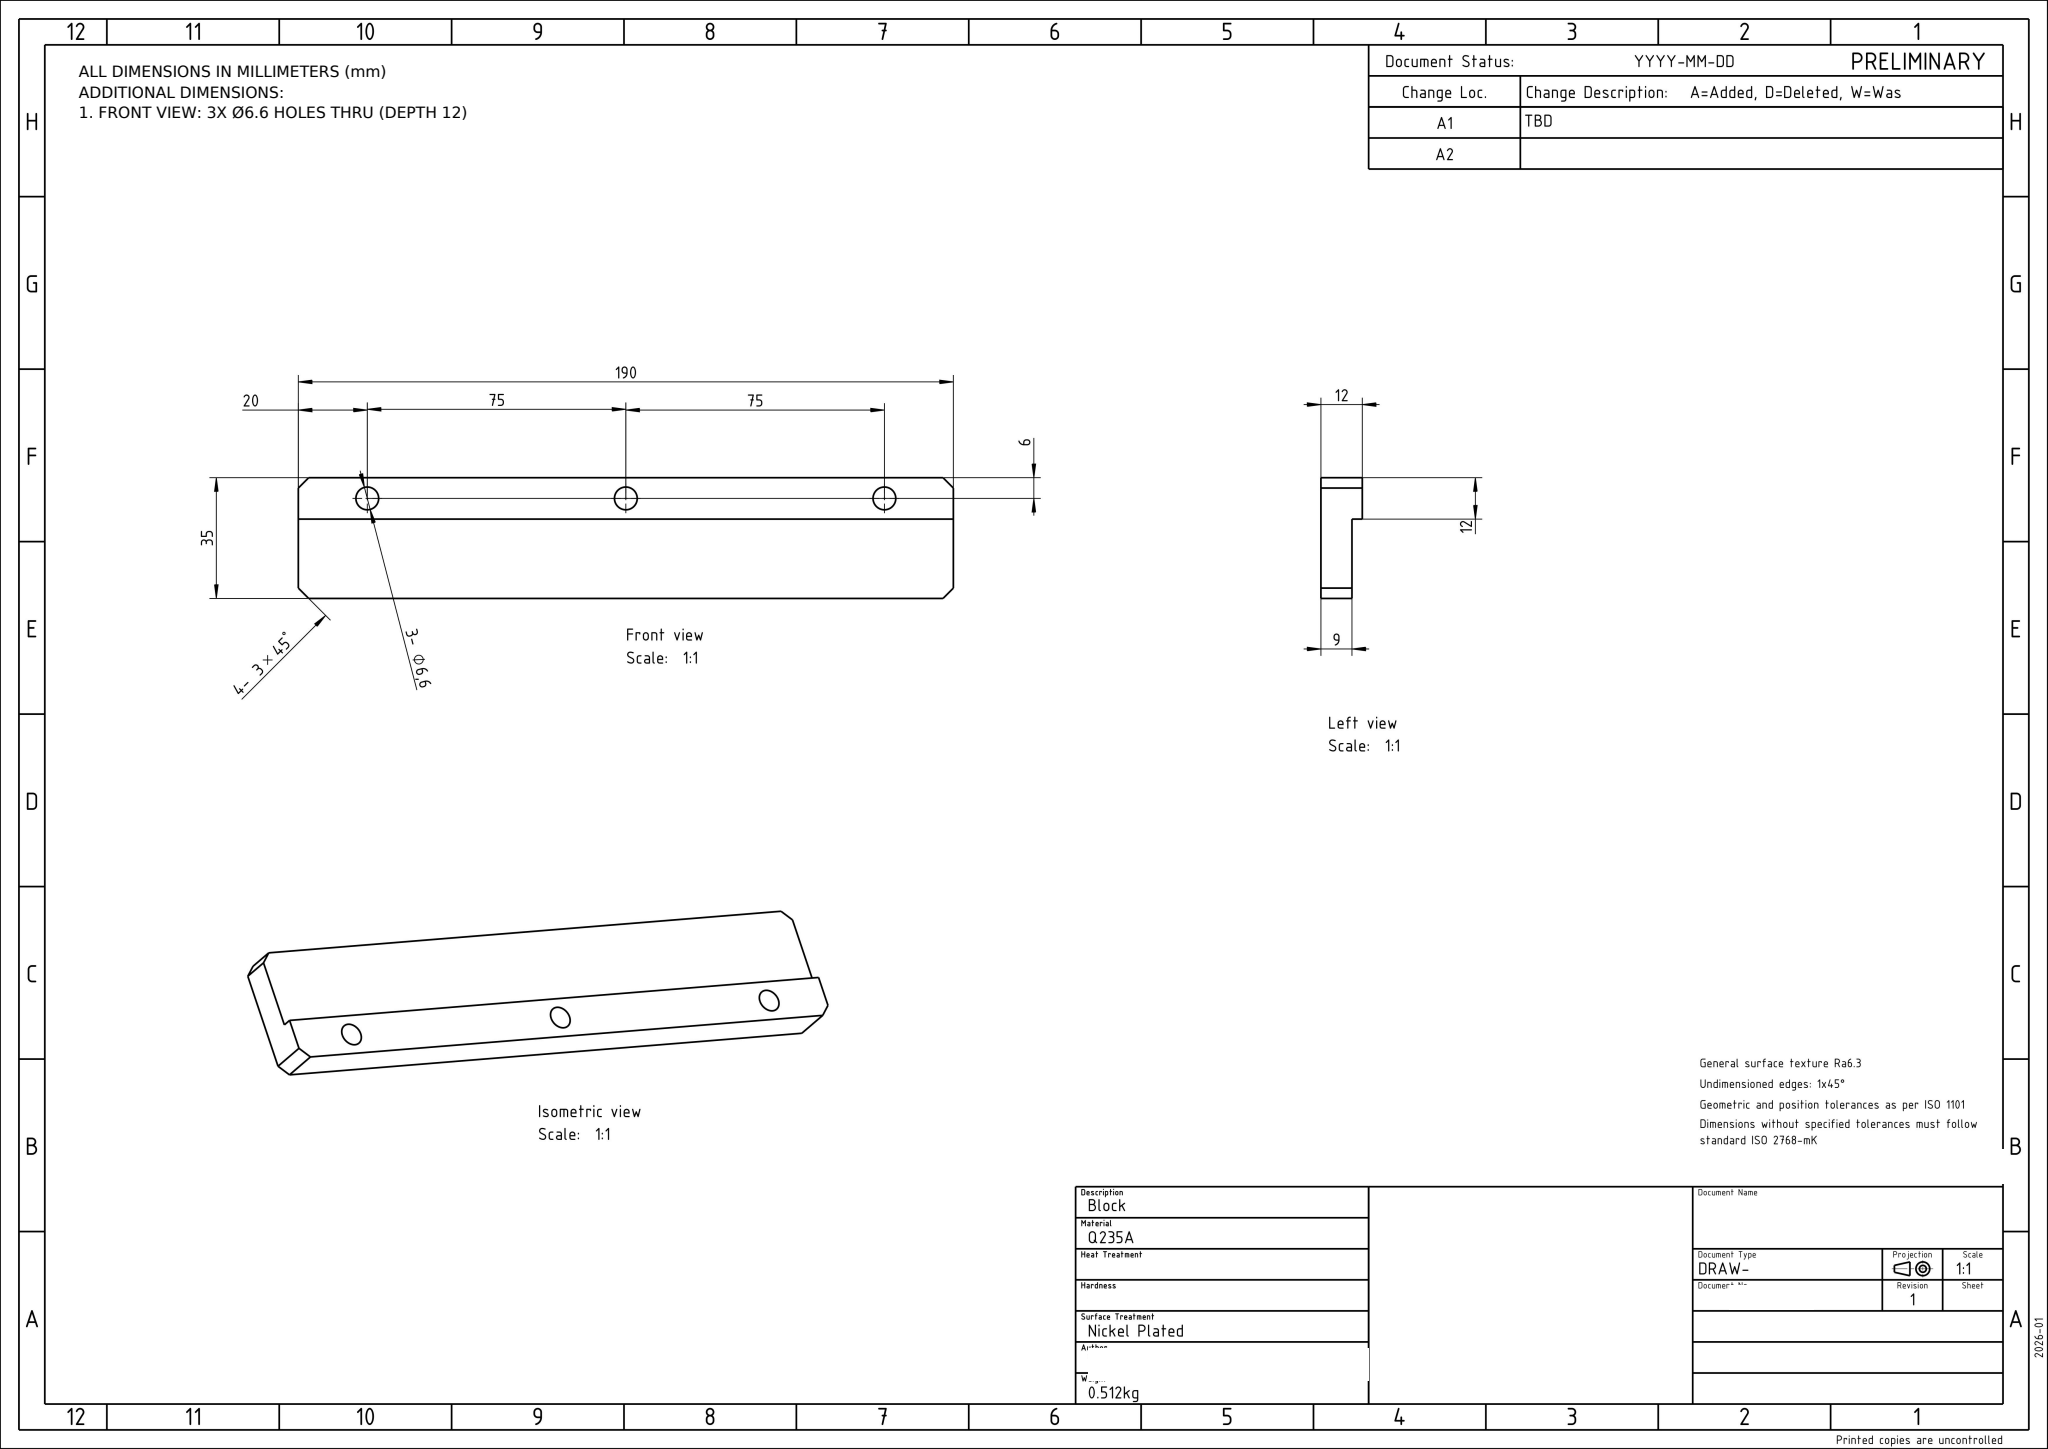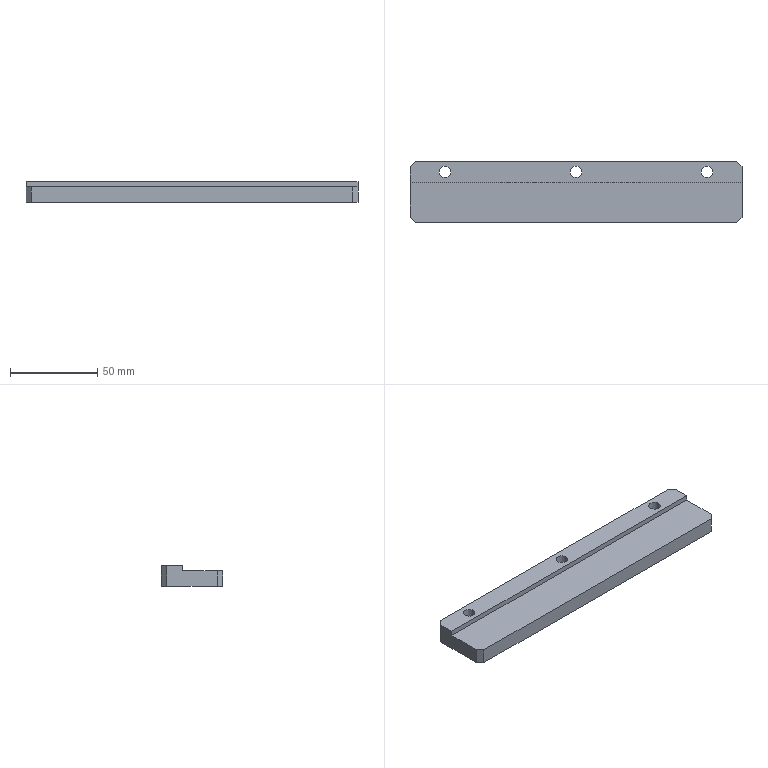Part | NX | mm | 1 solid | 15 faces | box 190 x 35 x 12 mm | volume 65269 mm3 | plane 12 | cylinder 3 | commonest cylinder face diameters 6.6 x3
STEP:
#1=CARTESIAN_POINT('',(0.,0.,0.));
#2=DIRECTION('',(0.,0.,1.));
#3=DIRECTION('',(1.,0.,0.));
#4=AXIS2_PLACEMENT_3D('',#1,#2,#3);
#5=(LENGTH_UNIT()NAMED_UNIT(*)SI_UNIT(.MILLI.,.METRE.));
#6=UNCERTAINTY_MEASURE_WITH_UNIT(LENGTH_MEASURE(0.00002),#5,'','');
#7=(NAMED_UNIT(*)PLANE_ANGLE_UNIT()SI_UNIT($,.RADIAN.));
#8=PLANE_ANGLE_MEASURE_WITH_UNIT(PLANE_ANGLE_MEASURE(0.01745),#7);
#9=DIMENSIONAL_EXPONENTS(0.,0.,0.,0.,0.,0.,0.);
#10=(CONVERSION_BASED_UNIT('',#8)NAMED_UNIT(#9)PLANE_ANGLE_UNIT());
#11=(NAMED_UNIT(*)SI_UNIT($,.STERADIAN.)SOLID_ANGLE_UNIT());
#12=(GEOMETRIC_REPRESENTATION_CONTEXT(3)GLOBAL_UNCERTAINTY_ASSIGNED_CONTEXT((#6))GLOBAL_UNIT_ASSIGNED_CONTEXT((#5,#10,#11))REPRESENTATION_CONTEXT('',''));
#13=SHAPE_REPRESENTATION('',(#4),#12);
#14=CARTESIAN_POINT('',(-95.,14.5,12.));
#15=VERTEX_POINT('',#14);
#16=CARTESIAN_POINT('',(-95.,5.5,12.));
#17=VERTEX_POINT('',#16);
#18=CARTESIAN_POINT('',(-95.,17.5,12.));
#19=DIRECTION('',(0.,-1.,0.));
#20=VECTOR('',#19,1.);
#21=LINE('',#18,#20);
#22=EDGE_CURVE('',#15,#17,#21,.T.);
#23=ORIENTED_EDGE('',*,*,#22,.F.);
#24=CARTESIAN_POINT('',(-95.,14.5,0.));
#25=VERTEX_POINT('',#24);
#26=CARTESIAN_POINT('',(-95.,14.5,9.));
#27=DIRECTION('',(0.,0.,-1.));
#28=VECTOR('',#27,1.);
#29=LINE('',#26,#28);
#30=EDGE_CURVE('',#15,#25,#29,.T.);
#31=ORIENTED_EDGE('',*,*,#30,.T.);
#32=CARTESIAN_POINT('',(-95.,-14.5,0.));
#33=VERTEX_POINT('',#32);
#34=CARTESIAN_POINT('',(-95.,17.5,0.));
#35=DIRECTION('',(0.,-1.,0.));
#36=VECTOR('',#35,1.);
#37=LINE('',#34,#36);
#38=EDGE_CURVE('',#25,#33,#37,.T.);
#39=ORIENTED_EDGE('',*,*,#38,.T.);
#40=CARTESIAN_POINT('',(-95.,-14.5,9.));
#41=VERTEX_POINT('',#40);
#42=CARTESIAN_POINT('',(-95.,-14.5,9.));
#43=DIRECTION('',(0.,0.,1.));
#44=VECTOR('',#43,1.);
#45=LINE('',#42,#44);
#46=EDGE_CURVE('',#33,#41,#45,.T.);
#47=ORIENTED_EDGE('',*,*,#46,.T.);
#48=CARTESIAN_POINT('',(-95.,5.5,9.));
#49=VERTEX_POINT('',#48);
#50=CARTESIAN_POINT('',(-95.,17.5,9.));
#51=DIRECTION('',(0.,-1.,0.));
#52=VECTOR('',#51,1.);
#53=LINE('',#50,#52);
#54=EDGE_CURVE('',#49,#41,#53,.T.);
#55=ORIENTED_EDGE('',*,*,#54,.F.);
#56=CARTESIAN_POINT('',(-95.,5.5,9.));
#57=DIRECTION('',(0.,0.,1.));
#58=VECTOR('',#57,1.);
#59=LINE('',#56,#58);
#60=EDGE_CURVE('',#49,#17,#59,.T.);
#61=ORIENTED_EDGE('',*,*,#60,.T.);
#62=EDGE_LOOP('',(#23,#31,#39,#47,#55,#61));
#63=FACE_OUTER_BOUND('',#62,.T.);
#64=CARTESIAN_POINT('',(-95.,17.5,9.));
#65=DIRECTION('',(1.,0.,0.));
#66=DIRECTION('',(-0.,1.,0.));
#67=AXIS2_PLACEMENT_3D('',#64,#65,#66);
#68=PLANE('',#67);
#69=ADVANCED_FACE('',(#63),#68,.F.);
#70=CARTESIAN_POINT('',(-92.,-17.5,0.));
#71=VERTEX_POINT('',#70);
#72=CARTESIAN_POINT('',(92.,-17.5,0.));
#73=VERTEX_POINT('',#72);
#74=CARTESIAN_POINT('',(-95.,-17.5,0.));
#75=DIRECTION('',(1.,0.,0.));
#76=VECTOR('',#75,1.);
#77=LINE('',#74,#76);
#78=EDGE_CURVE('',#71,#73,#77,.T.);
#79=ORIENTED_EDGE('',*,*,#78,.T.);
#80=CARTESIAN_POINT('',(92.,-17.5,9.));
#81=VERTEX_POINT('',#80);
#82=CARTESIAN_POINT('',(92.,-17.5,9.));
#83=DIRECTION('',(0.,0.,1.));
#84=VECTOR('',#83,1.);
#85=LINE('',#82,#84);
#86=EDGE_CURVE('',#73,#81,#85,.T.);
#87=ORIENTED_EDGE('',*,*,#86,.T.);
#88=CARTESIAN_POINT('',(-92.,-17.5,9.));
#89=VERTEX_POINT('',#88);
#90=CARTESIAN_POINT('',(-95.,-17.5,9.));
#91=DIRECTION('',(1.,0.,0.));
#92=VECTOR('',#91,1.);
#93=LINE('',#90,#92);
#94=EDGE_CURVE('',#89,#81,#93,.T.);
#95=ORIENTED_EDGE('',*,*,#94,.F.);
#96=CARTESIAN_POINT('',(-92.,-17.5,9.));
#97=DIRECTION('',(0.,0.,-1.));
#98=VECTOR('',#97,1.);
#99=LINE('',#96,#98);
#100=EDGE_CURVE('',#89,#71,#99,.T.);
#101=ORIENTED_EDGE('',*,*,#100,.T.);
#102=EDGE_LOOP('',(#79,#87,#95,#101));
#103=FACE_OUTER_BOUND('',#102,.T.);
#104=CARTESIAN_POINT('',(-95.,-17.5,9.));
#105=DIRECTION('',(0.,1.,0.));
#106=DIRECTION('',(0.,0.,1.));
#107=AXIS2_PLACEMENT_3D('',#104,#105,#106);
#108=PLANE('',#107);
#109=ADVANCED_FACE('',(#103),#108,.F.);
#110=CARTESIAN_POINT('',(95.,-14.5,0.));
#111=VERTEX_POINT('',#110);
#112=CARTESIAN_POINT('',(95.,14.5,0.));
#113=VERTEX_POINT('',#112);
#114=CARTESIAN_POINT('',(95.,-17.5,0.));
#115=DIRECTION('',(-0.,1.,0.));
#116=VECTOR('',#115,1.);
#117=LINE('',#114,#116);
#118=EDGE_CURVE('',#111,#113,#117,.T.);
#119=ORIENTED_EDGE('',*,*,#118,.T.);
#120=CARTESIAN_POINT('',(95.,14.5,12.));
#121=VERTEX_POINT('',#120);
#122=CARTESIAN_POINT('',(95.,14.5,9.));
#123=DIRECTION('',(0.,0.,1.));
#124=VECTOR('',#123,1.);
#125=LINE('',#122,#124);
#126=EDGE_CURVE('',#113,#121,#125,.T.);
#127=ORIENTED_EDGE('',*,*,#126,.T.);
#128=CARTESIAN_POINT('',(95.,5.5,12.));
#129=VERTEX_POINT('',#128);
#130=CARTESIAN_POINT('',(95.,17.5,12.));
#131=DIRECTION('',(0.,-1.,0.));
#132=VECTOR('',#131,1.);
#133=LINE('',#130,#132);
#134=EDGE_CURVE('',#121,#129,#133,.T.);
#135=ORIENTED_EDGE('',*,*,#134,.T.);
#136=CARTESIAN_POINT('',(95.,5.5,9.));
#137=VERTEX_POINT('',#136);
#138=CARTESIAN_POINT('',(95.,5.5,9.));
#139=DIRECTION('',(0.,0.,1.));
#140=VECTOR('',#139,1.);
#141=LINE('',#138,#140);
#142=EDGE_CURVE('',#137,#129,#141,.T.);
#143=ORIENTED_EDGE('',*,*,#142,.F.);
#144=CARTESIAN_POINT('',(95.,-14.5,9.));
#145=VERTEX_POINT('',#144);
#146=CARTESIAN_POINT('',(95.,-17.5,9.));
#147=DIRECTION('',(-0.,1.,0.));
#148=VECTOR('',#147,1.);
#149=LINE('',#146,#148);
#150=EDGE_CURVE('',#145,#137,#149,.T.);
#151=ORIENTED_EDGE('',*,*,#150,.F.);
#152=CARTESIAN_POINT('',(95.,-14.5,9.));
#153=DIRECTION('',(0.,0.,-1.));
#154=VECTOR('',#153,1.);
#155=LINE('',#152,#154);
#156=EDGE_CURVE('',#145,#111,#155,.T.);
#157=ORIENTED_EDGE('',*,*,#156,.T.);
#158=EDGE_LOOP('',(#119,#127,#135,#143,#151,#157));
#159=FACE_OUTER_BOUND('',#158,.T.);
#160=CARTESIAN_POINT('',(95.,-17.5,9.));
#161=DIRECTION('',(-1.,-0.,0.));
#162=DIRECTION('',(0.,-1.,0.));
#163=AXIS2_PLACEMENT_3D('',#160,#161,#162);
#164=PLANE('',#163);
#165=ADVANCED_FACE('',(#159),#164,.F.);
#166=CARTESIAN_POINT('',(92.,17.5,0.));
#167=VERTEX_POINT('',#166);
#168=CARTESIAN_POINT('',(-92.,17.5,0.));
#169=VERTEX_POINT('',#168);
#170=CARTESIAN_POINT('',(95.,17.5,0.));
#171=DIRECTION('',(-1.,0.,0.));
#172=VECTOR('',#171,1.);
#173=LINE('',#170,#172);
#174=EDGE_CURVE('',#167,#169,#173,.T.);
#175=ORIENTED_EDGE('',*,*,#174,.T.);
#176=CARTESIAN_POINT('',(-92.,17.5,12.));
#177=VERTEX_POINT('',#176);
#178=CARTESIAN_POINT('',(-92.,17.5,9.));
#179=DIRECTION('',(0.,0.,1.));
#180=VECTOR('',#179,1.);
#181=LINE('',#178,#180);
#182=EDGE_CURVE('',#169,#177,#181,.T.);
#183=ORIENTED_EDGE('',*,*,#182,.T.);
#184=CARTESIAN_POINT('',(92.,17.5,12.));
#185=VERTEX_POINT('',#184);
#186=CARTESIAN_POINT('',(-95.,17.5,12.));
#187=DIRECTION('',(1.,0.,0.));
#188=VECTOR('',#187,1.);
#189=LINE('',#186,#188);
#190=EDGE_CURVE('',#177,#185,#189,.T.);
#191=ORIENTED_EDGE('',*,*,#190,.T.);
#192=CARTESIAN_POINT('',(92.,17.5,9.));
#193=DIRECTION('',(0.,0.,-1.));
#194=VECTOR('',#193,1.);
#195=LINE('',#192,#194);
#196=EDGE_CURVE('',#185,#167,#195,.T.);
#197=ORIENTED_EDGE('',*,*,#196,.T.);
#198=EDGE_LOOP('',(#175,#183,#191,#197));
#199=FACE_OUTER_BOUND('',#198,.T.);
#200=CARTESIAN_POINT('',(95.,17.5,9.));
#201=DIRECTION('',(0.,-1.,0.));
#202=DIRECTION('',(0.,0.,-1.));
#203=AXIS2_PLACEMENT_3D('',#200,#201,#202);
#204=PLANE('',#203);
#205=ADVANCED_FACE('',(#199),#204,.F.);
#206=ORIENTED_EDGE('',*,*,#94,.T.);
#207=CARTESIAN_POINT('',(54.75,-54.75,9.));
#208=DIRECTION('',(0.7071,0.7071,0.));
#209=VECTOR('',#208,1.);
#210=LINE('',#207,#209);
#211=EDGE_CURVE('',#81,#145,#210,.T.);
#212=ORIENTED_EDGE('',*,*,#211,.T.);
#213=ORIENTED_EDGE('',*,*,#150,.T.);
#214=CARTESIAN_POINT('',(-95.,5.5,9.));
#215=DIRECTION('',(1.,0.,0.));
#216=VECTOR('',#215,1.);
#217=LINE('',#214,#216);
#218=EDGE_CURVE('',#49,#137,#217,.T.);
#219=ORIENTED_EDGE('',*,*,#218,.F.);
#220=ORIENTED_EDGE('',*,*,#54,.T.);
#221=CARTESIAN_POINT('',(-54.75,-54.75,9.));
#222=DIRECTION('',(0.7071,-0.7071,0.));
#223=VECTOR('',#222,1.);
#224=LINE('',#221,#223);
#225=EDGE_CURVE('',#41,#89,#224,.T.);
#226=ORIENTED_EDGE('',*,*,#225,.T.);
#227=EDGE_LOOP('',(#206,#212,#213,#219,#220,#226));
#228=FACE_OUTER_BOUND('',#227,.T.);
#229=CARTESIAN_POINT('',(0.,0.,9.));
#230=DIRECTION('',(0.,0.,1.));
#231=DIRECTION('',(1.,0.,0.));
#232=AXIS2_PLACEMENT_3D('',#229,#230,#231);
#233=PLANE('',#232);
#234=ADVANCED_FACE('',(#228),#233,.T.);
#235=CARTESIAN_POINT('',(78.3,11.5,0.));
#236=VERTEX_POINT('',#235);
#237=CARTESIAN_POINT('',(75.,11.5,0.));
#238=DIRECTION('',(0.,0.,1.));
#239=DIRECTION('',(1.,0.,0.));
#240=AXIS2_PLACEMENT_3D('',#237,#238,#239);
#241=CIRCLE('',#240,3.3);
#242=EDGE_CURVE('',#236,#236,#241,.T.);
#243=ORIENTED_EDGE('',*,*,#242,.T.);
#244=EDGE_LOOP('',(#243));
#245=FACE_BOUND('',#244,.T.);
#246=CARTESIAN_POINT('',(3.3,11.5,0.));
#247=VERTEX_POINT('',#246);
#248=CARTESIAN_POINT('',(0.,11.5,0.));
#249=DIRECTION('',(0.,0.,1.));
#250=DIRECTION('',(1.,0.,0.));
#251=AXIS2_PLACEMENT_3D('',#248,#249,#250);
#252=CIRCLE('',#251,3.3);
#253=EDGE_CURVE('',#247,#247,#252,.T.);
#254=ORIENTED_EDGE('',*,*,#253,.T.);
#255=EDGE_LOOP('',(#254));
#256=FACE_BOUND('',#255,.T.);
#257=CARTESIAN_POINT('',(-71.7,11.5,0.));
#258=VERTEX_POINT('',#257);
#259=CARTESIAN_POINT('',(-75.,11.5,0.));
#260=DIRECTION('',(0.,0.,1.));
#261=DIRECTION('',(1.,0.,0.));
#262=AXIS2_PLACEMENT_3D('',#259,#260,#261);
#263=CIRCLE('',#262,3.3);
#264=EDGE_CURVE('',#258,#258,#263,.T.);
#265=ORIENTED_EDGE('',*,*,#264,.T.);
#266=EDGE_LOOP('',(#265));
#267=FACE_BOUND('',#266,.T.);
#268=ORIENTED_EDGE('',*,*,#38,.F.);
#269=CARTESIAN_POINT('',(-95.,14.5,0.));
#270=DIRECTION('',(0.7071,0.7071,0.));
#271=VECTOR('',#270,1.);
#272=LINE('',#269,#271);
#273=EDGE_CURVE('',#25,#169,#272,.T.);
#274=ORIENTED_EDGE('',*,*,#273,.T.);
#275=ORIENTED_EDGE('',*,*,#174,.F.);
#276=CARTESIAN_POINT('',(92.,17.5,0.));
#277=DIRECTION('',(0.7071,-0.7071,0.));
#278=VECTOR('',#277,1.);
#279=LINE('',#276,#278);
#280=EDGE_CURVE('',#167,#113,#279,.T.);
#281=ORIENTED_EDGE('',*,*,#280,.T.);
#282=ORIENTED_EDGE('',*,*,#118,.F.);
#283=CARTESIAN_POINT('',(95.,-14.5,0.));
#284=DIRECTION('',(-0.7071,-0.7071,0.));
#285=VECTOR('',#284,1.);
#286=LINE('',#283,#285);
#287=EDGE_CURVE('',#111,#73,#286,.T.);
#288=ORIENTED_EDGE('',*,*,#287,.T.);
#289=ORIENTED_EDGE('',*,*,#78,.F.);
#290=CARTESIAN_POINT('',(-92.,-17.5,0.));
#291=DIRECTION('',(-0.7071,0.7071,0.));
#292=VECTOR('',#291,1.);
#293=LINE('',#290,#292);
#294=EDGE_CURVE('',#71,#33,#293,.T.);
#295=ORIENTED_EDGE('',*,*,#294,.T.);
#296=EDGE_LOOP('',(#268,#274,#275,#281,#282,#288,#289,#295));
#297=FACE_BOUND('',#296,.T.);
#298=CARTESIAN_POINT('',(0.,0.,0.));
#299=DIRECTION('',(0.,0.,1.));
#300=DIRECTION('',(1.,0.,0.));
#301=AXIS2_PLACEMENT_3D('',#298,#299,#300);
#302=PLANE('',#301);
#303=ADVANCED_FACE('',(#245,#256,#267,#297),#302,.F.);
#304=CARTESIAN_POINT('',(71.7,11.5,12.));
#305=VERTEX_POINT('',#304);
#306=CARTESIAN_POINT('',(75.,11.5,12.));
#307=DIRECTION('',(0.,0.,-1.));
#308=DIRECTION('',(-1.,0.,0.));
#309=AXIS2_PLACEMENT_3D('',#306,#307,#308);
#310=CIRCLE('',#309,3.3);
#311=EDGE_CURVE('',#305,#305,#310,.T.);
#312=ORIENTED_EDGE('',*,*,#311,.T.);
#313=EDGE_LOOP('',(#312));
#314=FACE_BOUND('',#313,.T.);
#315=CARTESIAN_POINT('',(-3.3,11.5,12.));
#316=VERTEX_POINT('',#315);
#317=CARTESIAN_POINT('',(0.,11.5,12.));
#318=DIRECTION('',(0.,0.,-1.));
#319=DIRECTION('',(-1.,0.,0.));
#320=AXIS2_PLACEMENT_3D('',#317,#318,#319);
#321=CIRCLE('',#320,3.3);
#322=EDGE_CURVE('',#316,#316,#321,.T.);
#323=ORIENTED_EDGE('',*,*,#322,.T.);
#324=EDGE_LOOP('',(#323));
#325=FACE_BOUND('',#324,.T.);
#326=CARTESIAN_POINT('',(-78.3,11.5,12.));
#327=VERTEX_POINT('',#326);
#328=CARTESIAN_POINT('',(-75.,11.5,12.));
#329=DIRECTION('',(0.,0.,-1.));
#330=DIRECTION('',(-1.,0.,0.));
#331=AXIS2_PLACEMENT_3D('',#328,#329,#330);
#332=CIRCLE('',#331,3.3);
#333=EDGE_CURVE('',#327,#327,#332,.T.);
#334=ORIENTED_EDGE('',*,*,#333,.T.);
#335=EDGE_LOOP('',(#334));
#336=FACE_BOUND('',#335,.T.);
#337=ORIENTED_EDGE('',*,*,#190,.F.);
#338=CARTESIAN_POINT('',(-93.5,16.,12.));
#339=DIRECTION('',(-0.7071,-0.7071,0.));
#340=VECTOR('',#339,1.);
#341=LINE('',#338,#340);
#342=EDGE_CURVE('',#177,#15,#341,.T.);
#343=ORIENTED_EDGE('',*,*,#342,.T.);
#344=ORIENTED_EDGE('',*,*,#22,.T.);
#345=CARTESIAN_POINT('',(-95.,5.5,12.));
#346=DIRECTION('',(1.,0.,0.));
#347=VECTOR('',#346,1.);
#348=LINE('',#345,#347);
#349=EDGE_CURVE('',#17,#129,#348,.T.);
#350=ORIENTED_EDGE('',*,*,#349,.T.);
#351=ORIENTED_EDGE('',*,*,#134,.F.);
#352=CARTESIAN_POINT('',(-1.5,111.,12.));
#353=DIRECTION('',(-0.7071,0.7071,0.));
#354=VECTOR('',#353,1.);
#355=LINE('',#352,#354);
#356=EDGE_CURVE('',#121,#185,#355,.T.);
#357=ORIENTED_EDGE('',*,*,#356,.T.);
#358=EDGE_LOOP('',(#337,#343,#344,#350,#351,#357));
#359=FACE_BOUND('',#358,.T.);
#360=CARTESIAN_POINT('',(-95.,17.5,12.));
#361=DIRECTION('',(0.,0.,-1.));
#362=DIRECTION('',(1.,0.,0.));
#363=AXIS2_PLACEMENT_3D('',#360,#361,#362);
#364=PLANE('',#363);
#365=ADVANCED_FACE('',(#314,#325,#336,#359),#364,.F.);
#366=ORIENTED_EDGE('',*,*,#349,.F.);
#367=ORIENTED_EDGE('',*,*,#60,.F.);
#368=ORIENTED_EDGE('',*,*,#218,.T.);
#369=ORIENTED_EDGE('',*,*,#142,.T.);
#370=EDGE_LOOP('',(#366,#367,#368,#369));
#371=FACE_OUTER_BOUND('',#370,.T.);
#372=CARTESIAN_POINT('',(-95.,5.5,9.));
#373=DIRECTION('',(0.,-1.,0.));
#374=DIRECTION('',(0.,0.,-1.));
#375=AXIS2_PLACEMENT_3D('',#372,#373,#374);
#376=PLANE('',#375);
#377=ADVANCED_FACE('',(#371),#376,.T.);
#378=ORIENTED_EDGE('',*,*,#333,.F.);
#379=EDGE_LOOP('',(#378));
#380=FACE_BOUND('',#379,.T.);
#381=ORIENTED_EDGE('',*,*,#264,.F.);
#382=EDGE_LOOP('',(#381));
#383=FACE_BOUND('',#382,.T.);
#384=CARTESIAN_POINT('',(-75.,11.5,12.));
#385=DIRECTION('',(0.,0.,-1.));
#386=DIRECTION('',(-1.,0.,0.));
#387=AXIS2_PLACEMENT_3D('',#384,#385,#386);
#388=CYLINDRICAL_SURFACE('',#387,3.3);
#389=ADVANCED_FACE('',(#380,#383),#388,.F.);
#390=ORIENTED_EDGE('',*,*,#322,.F.);
#391=EDGE_LOOP('',(#390));
#392=FACE_BOUND('',#391,.T.);
#393=ORIENTED_EDGE('',*,*,#253,.F.);
#394=EDGE_LOOP('',(#393));
#395=FACE_BOUND('',#394,.T.);
#396=CARTESIAN_POINT('',(0.,11.5,12.));
#397=DIRECTION('',(0.,0.,-1.));
#398=DIRECTION('',(-1.,0.,0.));
#399=AXIS2_PLACEMENT_3D('',#396,#397,#398);
#400=CYLINDRICAL_SURFACE('',#399,3.3);
#401=ADVANCED_FACE('',(#392,#395),#400,.F.);
#402=ORIENTED_EDGE('',*,*,#311,.F.);
#403=EDGE_LOOP('',(#402));
#404=FACE_BOUND('',#403,.T.);
#405=ORIENTED_EDGE('',*,*,#242,.F.);
#406=EDGE_LOOP('',(#405));
#407=FACE_BOUND('',#406,.T.);
#408=CARTESIAN_POINT('',(75.,11.5,12.));
#409=DIRECTION('',(0.,0.,-1.));
#410=DIRECTION('',(-1.,0.,0.));
#411=AXIS2_PLACEMENT_3D('',#408,#409,#410);
#412=CYLINDRICAL_SURFACE('',#411,3.3);
#413=ADVANCED_FACE('',(#404,#407),#412,.F.);
#414=ORIENTED_EDGE('',*,*,#342,.F.);
#415=ORIENTED_EDGE('',*,*,#182,.F.);
#416=ORIENTED_EDGE('',*,*,#273,.F.);
#417=ORIENTED_EDGE('',*,*,#30,.F.);
#418=EDGE_LOOP('',(#414,#415,#416,#417));
#419=FACE_OUTER_BOUND('',#418,.T.);
#420=CARTESIAN_POINT('',(-95.,14.5,9.));
#421=DIRECTION('',(0.7071,-0.7071,0.));
#422=DIRECTION('',(0.,0.,-1.));
#423=AXIS2_PLACEMENT_3D('',#420,#421,#422);
#424=PLANE('',#423);
#425=ADVANCED_FACE('',(#419),#424,.F.);
#426=ORIENTED_EDGE('',*,*,#356,.F.);
#427=ORIENTED_EDGE('',*,*,#126,.F.);
#428=ORIENTED_EDGE('',*,*,#280,.F.);
#429=ORIENTED_EDGE('',*,*,#196,.F.);
#430=EDGE_LOOP('',(#426,#427,#428,#429));
#431=FACE_OUTER_BOUND('',#430,.T.);
#432=CARTESIAN_POINT('',(92.,17.5,9.));
#433=DIRECTION('',(-0.7071,-0.7071,0.));
#434=DIRECTION('',(0.,0.,-1.));
#435=AXIS2_PLACEMENT_3D('',#432,#433,#434);
#436=PLANE('',#435);
#437=ADVANCED_FACE('',(#431),#436,.F.);
#438=ORIENTED_EDGE('',*,*,#211,.F.);
#439=ORIENTED_EDGE('',*,*,#86,.F.);
#440=ORIENTED_EDGE('',*,*,#287,.F.);
#441=ORIENTED_EDGE('',*,*,#156,.F.);
#442=EDGE_LOOP('',(#438,#439,#440,#441));
#443=FACE_OUTER_BOUND('',#442,.T.);
#444=CARTESIAN_POINT('',(95.,-14.5,9.));
#445=DIRECTION('',(-0.7071,0.7071,0.));
#446=DIRECTION('',(0.,0.,-1.));
#447=AXIS2_PLACEMENT_3D('',#444,#445,#446);
#448=PLANE('',#447);
#449=ADVANCED_FACE('',(#443),#448,.F.);
#450=ORIENTED_EDGE('',*,*,#225,.F.);
#451=ORIENTED_EDGE('',*,*,#46,.F.);
#452=ORIENTED_EDGE('',*,*,#294,.F.);
#453=ORIENTED_EDGE('',*,*,#100,.F.);
#454=EDGE_LOOP('',(#450,#451,#452,#453));
#455=FACE_OUTER_BOUND('',#454,.T.);
#456=CARTESIAN_POINT('',(-92.,-17.5,9.));
#457=DIRECTION('',(0.7071,0.7071,0.));
#458=DIRECTION('',(0.,0.,-1.));
#459=AXIS2_PLACEMENT_3D('',#456,#457,#458);
#460=PLANE('',#459);
#461=ADVANCED_FACE('',(#455),#460,.F.);
#462=CLOSED_SHELL('',(#69,#109,#165,#205,#234,#303,#365,#377,#389,#401,#413,#425,#437,#449,#461));
#463=MANIFOLD_SOLID_BREP('',#462);
#464=ADVANCED_BREP_SHAPE_REPRESENTATION('',(#463),#12);
#465=SHAPE_REPRESENTATION_RELATIONSHIP('','',#13,#464);
#466=PRESENTATION_LAYER_ASSIGNMENT('','',(#463));
#467=COLOUR_RGB('',0.4,0.8,1.);
#468=FILL_AREA_STYLE_COLOUR('',#467);
#469=FILL_AREA_STYLE('',(#468));
#470=SURFACE_STYLE_FILL_AREA(#469);
#471=SURFACE_SIDE_STYLE('',(#470));
#472=SURFACE_STYLE_USAGE(.BOTH.,#471);
#473=PRESENTATION_STYLE_ASSIGNMENT((#472));
#474=STYLED_ITEM('',(#473),#463);
#475=MECHANICAL_DESIGN_GEOMETRIC_PRESENTATION_REPRESENTATION('',(#474),#12);